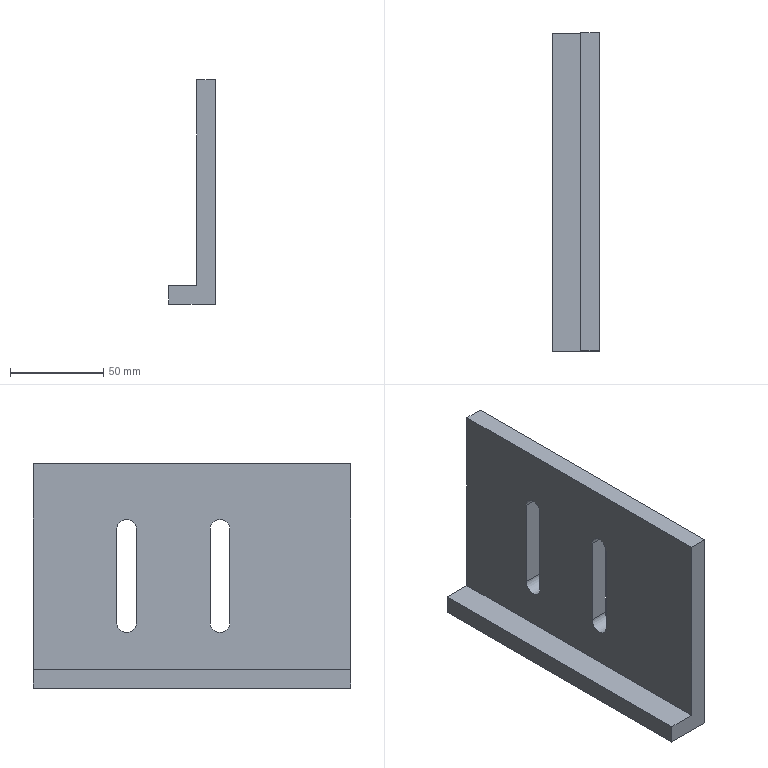Component | NX | FIXED_PLATE_3 | 1 solid | 16 faces | volume 217268 mm3 | plane 12 | cylinder 4 | commonest cylinder face diameters 10.5 x4